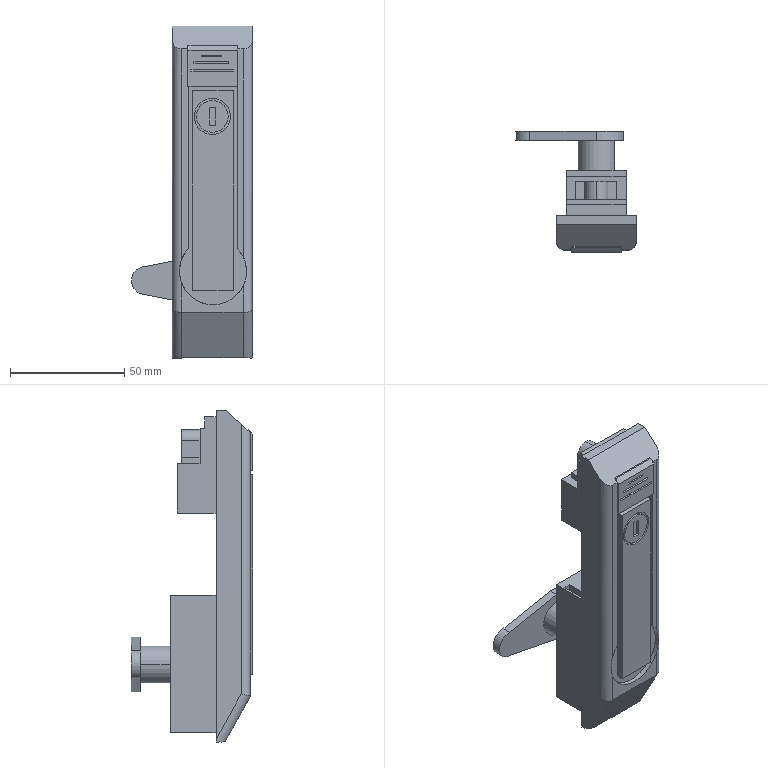Component | SolidWorks | GlassDoorAssembly-1_828LockAssembly-1_828LockHead-1 | 1 solid | 106 faces | volume 113904 mm3 | plane 82 | cylinder 24 | commonest cylinder face diameters 10 x6 8 x4 29.354 x3 23.767 x2 15.989 x2 13.835 x2 15.835 x2 6 x2